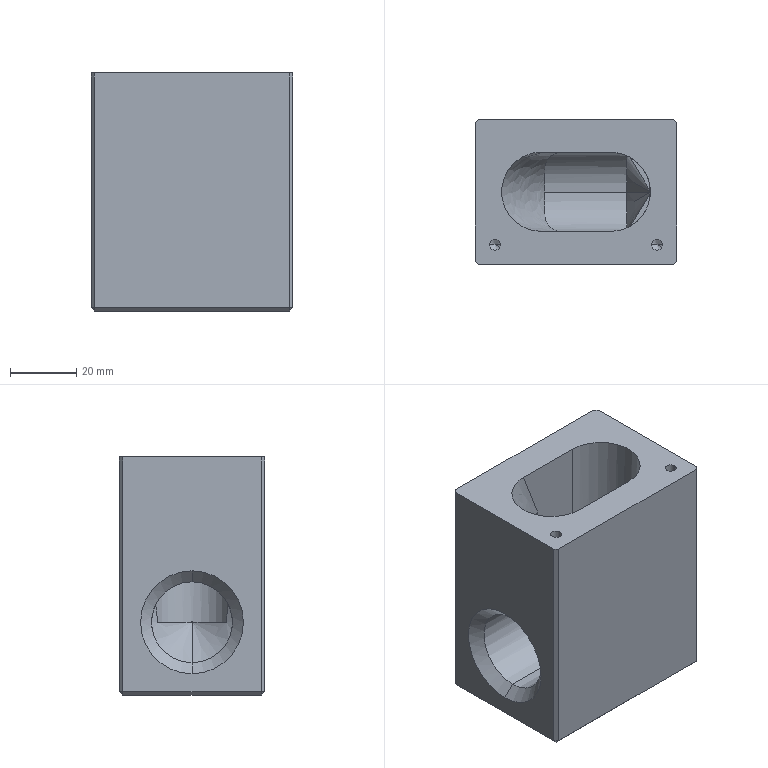CAM job | Mastercam | mm | 25 operations | part box 61 x 44 x 72
1. Facing | 1 - 50 J面铣
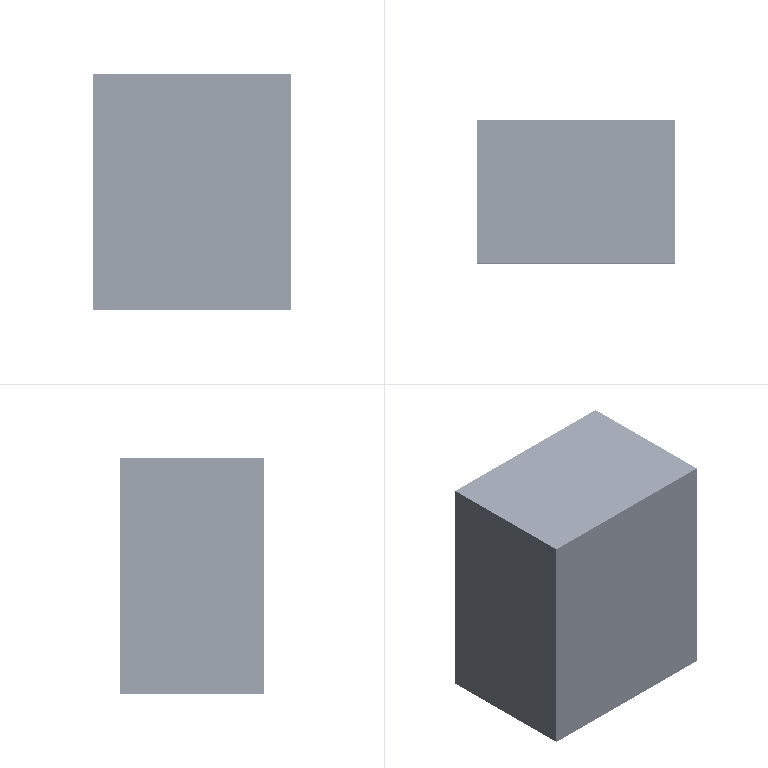2. 2D High Speed (2D Dynamic Mill) | 4 - 16.001 平铣刀C
3. Facing | 1 - 50 J面铣
4. Contour (2D) | 5 - 16 平铣刀J
5. Contour (2D chamfer) | 2 - 6定位倒角
6. Contour (2D chamfer) | 2 - 6定位倒角
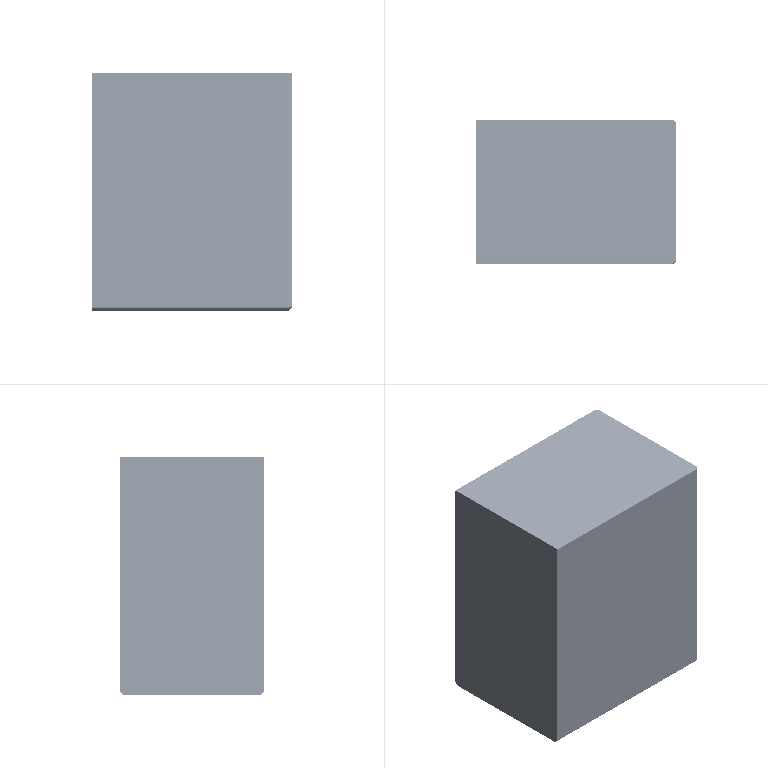7. Facing | 1 - 80 J面铣
8. Drill/Counterbore | 2 - 6定位倒角
9. Peck Drill | 23 - 24 钻头
10. Helix Bore | 4 - 16.001 平铣刀C
11. Contour (2D chamfer) | 2 - 6定位倒角
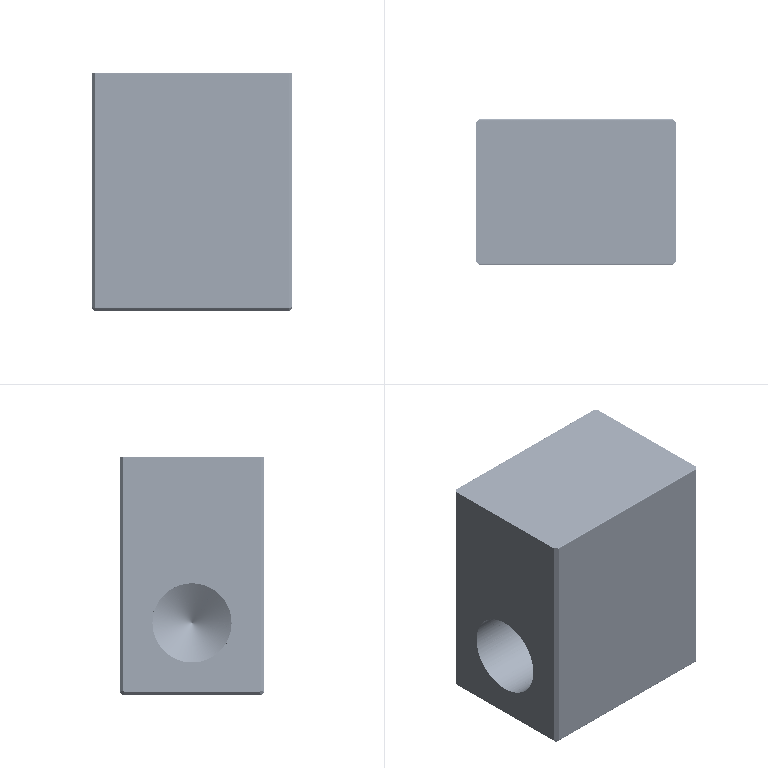12. Contour (2D chamfer) | 22 - 10 倒角刀
13. Thread Mill | 21 - 20.5 螺纹铣刀
14. Contour (2D chamfer) | 22 - 10 倒角刀
15. Facing | 1 - 80 J面铣
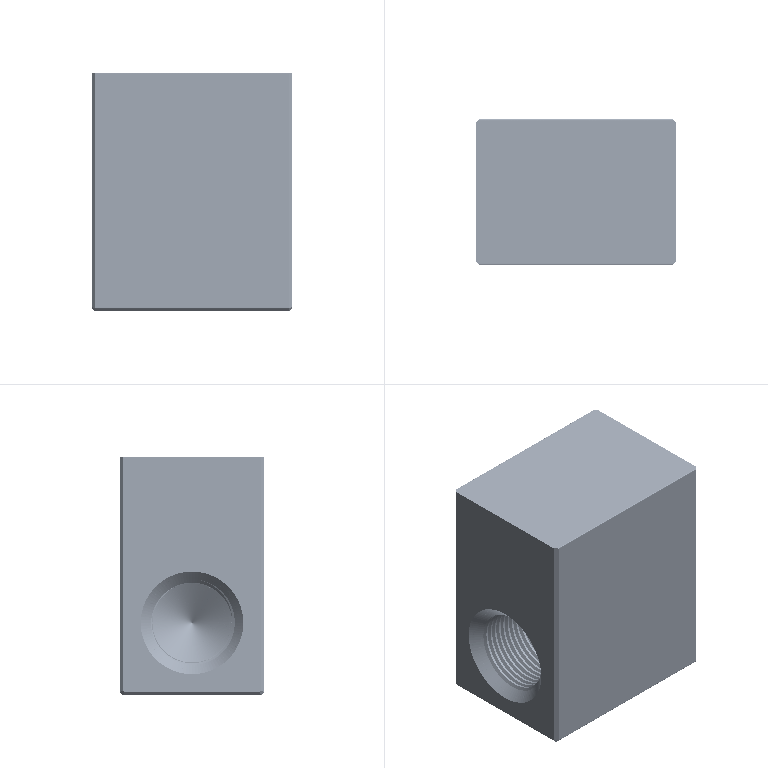16. 2D High Speed (2D Dynamic Mill) | 9 - 10C 平底刀
17. 3D High Speed (Waterline) | 4 - 16.001 平铣刀C
18. Contour (Remachining) | 11 - 8 J平底刀
19. Contour (2D) | 10 - 10J 平底刀
20. 3D High Speed (Waterline) | 3 - 10 -R1.0圆鼻铣刀
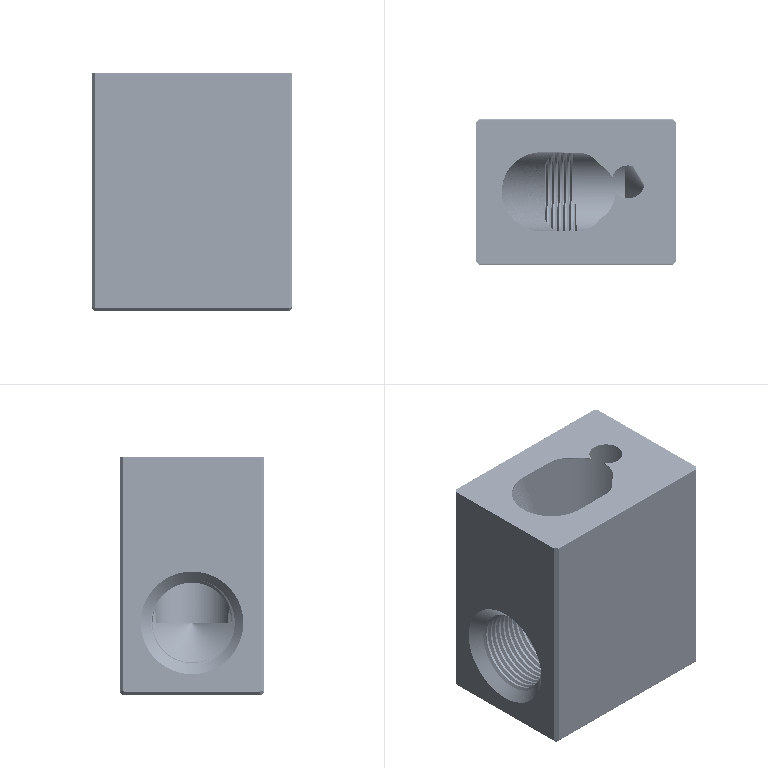21. Drill/Counterbore | 2 - 6定位倒角
22. Peck Drill | 12 - 3.3 钻头
23. Facing | 1 - 80 J面铣
24. Model Chamfer | 2 - 6定位倒角
25. Helix Bore | 24 - 2 平铣刀